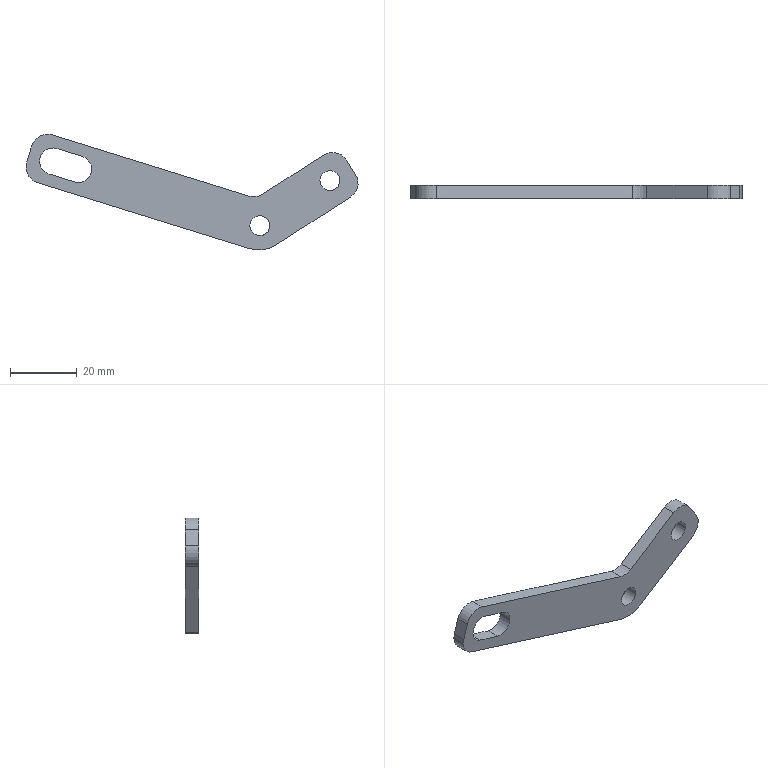Component | NX | LINK_3 | 1 solid | 20 faces | volume 5522 mm3 | plane 10 | cylinder 10 | commonest cylinder face diameters 10 x5 8 x2 6 x2 20 x1